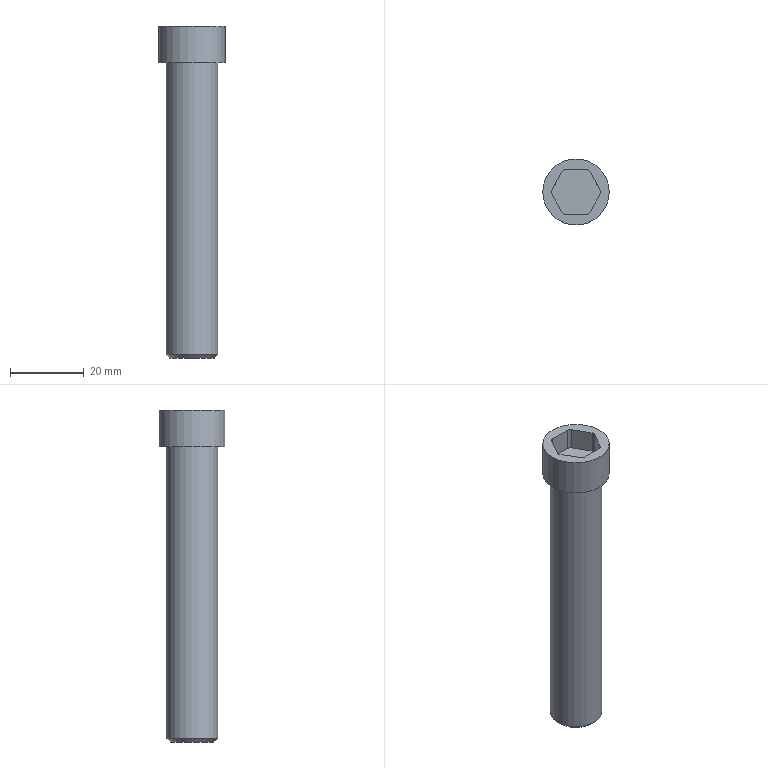Component | NX | SCREW_M14 | 1 solid | 19 faces | volume 14089 mm3 | plane 10 | cylinder 8 | cone 1 | commonest cylinder face diameters 2 x6 13.998 x1 18 x1